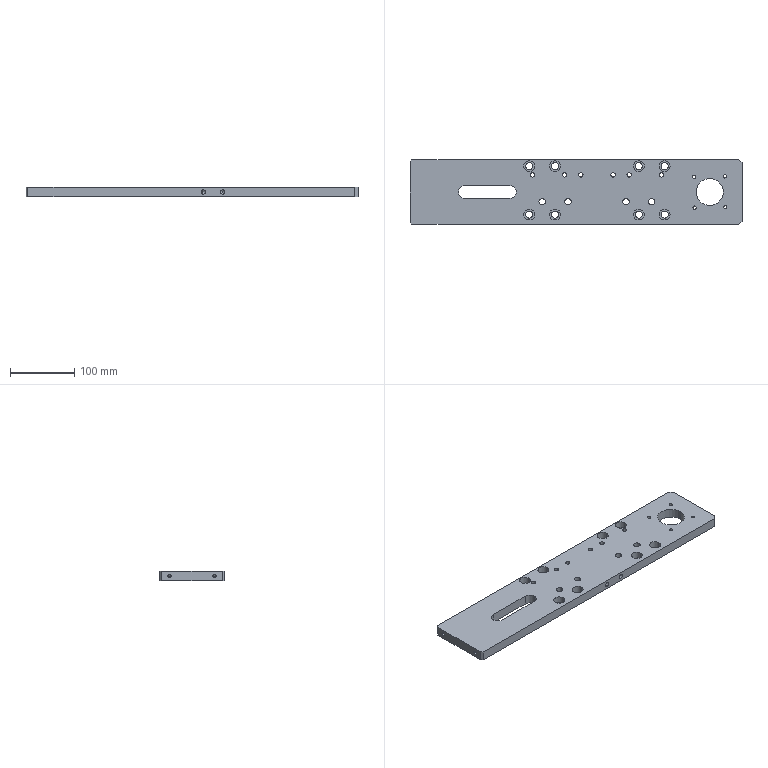Component | SolidWorks | -LowerSlideSleeveConnectionPlate02-1 | 1 solid | 101 faces | box 515 x 100 x 15 mm | volume 690969 mm3 | cylinder 73 | plane 20 | cone 8 | commonest cylinder face diameters 6.8 x16 17 x16 11 x16 5 x12 10 x8 20 x3 42 x2
build123d program:
from build123d import *

# Parameters (mm, degrees)
SKETCH1_W                                            = 555
SKETCH1_H                                            = 100
BOSS_EXTRUDE1_DEPTH                                  = 7.5
M10_TAPPED_HOLE1_D                                   = 10
CYLINDRICAL_COUNTERSUNK_HOLE_FOR_M10_HEX_D           = 11
CYLINDRICAL_COUNTERSUNK_HOLE_FOR_M10_HEX_CBORE_D     = 17
CYLINDRICAL_COUNTERSUNK_HOLE_FOR_M10_HEX_CBORE_DEPTH = 11
M8_TAPPED_HOLE1_D                                    = 6.8
SKETCH11_R                                           = 21
CUT_EXTRUDE1_DEPTH                                   = 15
M6_TAPPED_HOLE4_D                                    = 5
CIRPATTERN1_COUNT                                    = 4
CUT_EXTRUDE2_DEPTH                                   = 15
M6_TAPPED_HOLE3_D                                    = 5
M6_TAPPED_HOLE3_DEPTH                                = 17
M6_TAPPED_HOLE3_TIP                                  = 1.502
M10_TAPPED_HOLE2_D                                   = 10
CHAMFER1_SIZE                                        = 3
SKETCH23_W                                           = 40
SKETCH23_H                                           = 100
CUT_EXTRUDE3_DEPTH                                   = 283.367
CHAMFER2_SIZE                                        = 5
M8_TAPPED_HOLE2_D                                    = 6.8
M8_TAPPED_HOLE2_DEPTH                                = 22.25
M8_TAPPED_HOLE2_TIP                                  = 2.043


with BuildPart() as part:
    # Sketch1 → Boss-Extrude1 (new, symmetric)
    with BuildSketch(Plane.XY):
        Rectangle(SKETCH1_W, SKETCH1_H)
    extrude(amount=BOSS_EXTRUDE1_DEPTH, both=True)

    # M10 Tapped Hole1 (through all)
    with Locations(Plane(origin=(0, 0, -7.5), x_dir=(1, 0, 0), z_dir=(0, 0, -1))):
        with Locations((97.5, 15), (-72.5, 15)):
            Hole(M10_TAPPED_HOLE1_D / 2)

    # Cylindrical Countersunk Hole for M10 Hex (through all)
    with Locations(Plane.XY.offset(7.5)):
        with Locations((117.5, 40), (117.5, -35), (77.5, 40), (77.5, -35), (-52.5, -35), (-92.5, -35), (-92.5, 40), (-52.5, 40)):
            CounterBoreHole(CYLINDRICAL_COUNTERSUNK_HOLE_FOR_M10_HEX_D / 2, CYLINDRICAL_COUNTERSUNK_HOLE_FOR_M10_HEX_CBORE_D / 2, CYLINDRICAL_COUNTERSUNK_HOLE_FOR_M10_HEX_CBORE_DEPTH)

    # M8 Tapped Hole1 (through all)
    with Locations(Plane.XY.offset(7.5)):
        with Locations((112.5, 26.5), (62.5, 26.5), (37.5, 26.5), (-12.5, 26.5), (-37.5, 26.5), (-87.5, 26.5)):
            Hole(M8_TAPPED_HOLE1_D / 2)

    # Sketch11 → Cut-Extrude1 (cut)
    with BuildSketch(Plane.XY.offset(7.5)):
        with Locations((187.5, 0)):
            Circle(SKETCH11_R)
    extrude(amount=-CUT_EXTRUDE1_DEPTH, mode=Mode.SUBTRACT)

    # M6 Tapped Hole4 (through all)
    with Locations(Plane.XY.offset(7.5)):
        with Locations((163.315, 23.54)):
            m6_tapped_hole4 = Hole(M6_TAPPED_HOLE4_D / 2)

    # CirPattern1: M6 Tapped Hole4 ×4 about axis
    cirpattern1_axis = Axis((187.5, 0, 0), (0, 0, 1))
    for i in range(1, CIRPATTERN1_COUNT):
        add(m6_tapped_hole4.rotate(cirpattern1_axis, i * 360 / CIRPATTERN1_COUNT), mode=Mode.SUBTRACT)

    # Sketch14 → Cut-Extrude2 (cut)
    with BuildSketch(Plane.XY.offset(7.5)):
        with BuildLine():
            Line((-192.5, 10), (-122.5, 10))
            ThreePointArc((-122.5, 10), (-112.5, 0), (-122.5, -10))
            Line((-122.5, -10), (-192.5, -10))
            ThreePointArc((-192.5, -10), (-202.5, 0), (-192.5, 10))
        make_face()
    extrude(amount=-CUT_EXTRUDE2_DEPTH, mode=Mode.SUBTRACT)

    # M6 Tapped Hole3
    with Locations(Plane.ZY.offset(277.5)):
        with Locations((0, 35), (0, -35)):
            Hole(M6_TAPPED_HOLE3_D / 2, depth=M6_TAPPED_HOLE3_DEPTH)
            with Locations((0, 0, -(M6_TAPPED_HOLE3_DEPTH + M6_TAPPED_HOLE3_TIP / 2))):  # 118° drill point
                Cone(0, M6_TAPPED_HOLE3_D / 2, M6_TAPPED_HOLE3_TIP, mode=Mode.SUBTRACT)

    # M10 Tapped Hole2 (through all)
    with Locations(Plane(origin=(0, 0, -7.5), x_dir=(-1, 0, 0), z_dir=(0, 0, -1))):
        with Locations((-57.5, -15), (32.5, -15)):
            Hole(M10_TAPPED_HOLE2_D / 2)

    # Chamfer1
    chamfer1_edges = [part.edges().sort_by_distance(p)[0] for p in [
        (277.5, -50, 0),
        (-277.5, -50, 0),
        (-277.5, 50, 0),
        (277.5, 50, 0),
    ]]
    chamfer(chamfer1_edges, length=CHAMFER1_SIZE)

    # Sketch23 → Cut-Extrude3 (cut, through all)
    with BuildSketch(Plane(origin=(0, 0, -7.5), x_dir=(-1, 0, 0), z_dir=(0, 0, -1))):
        with Locations((-257.5, 0)):
            Rectangle(SKETCH23_W, SKETCH23_H)
    extrude(amount=-CUT_EXTRUDE3_DEPTH, mode=Mode.SUBTRACT)

    # Chamfer2
    chamfer2_edges = [part.edges().sort_by_distance(p)[0] for p in [
        (237.5, 50, 0),
        (237.5, -50, 0),
    ]]
    chamfer(chamfer2_edges, length=CHAMFER2_SIZE)

    # M8 Tapped Hole2
    with Locations(Plane.XZ.offset(50)):
        with Locations((-2.5, 0), (27.5, 0)):
            Hole(M8_TAPPED_HOLE2_D / 2, depth=M8_TAPPED_HOLE2_DEPTH)
            with Locations((0, 0, -(M8_TAPPED_HOLE2_DEPTH + M8_TAPPED_HOLE2_TIP / 2))):  # 118° drill point
                Cone(0, M8_TAPPED_HOLE2_D / 2, M8_TAPPED_HOLE2_TIP, mode=Mode.SUBTRACT)


solid = part.part

# Placed as in the assembly
solid = solid.moved(Location((17.5, 1094.5, -2.5), (0, 0, 0)))